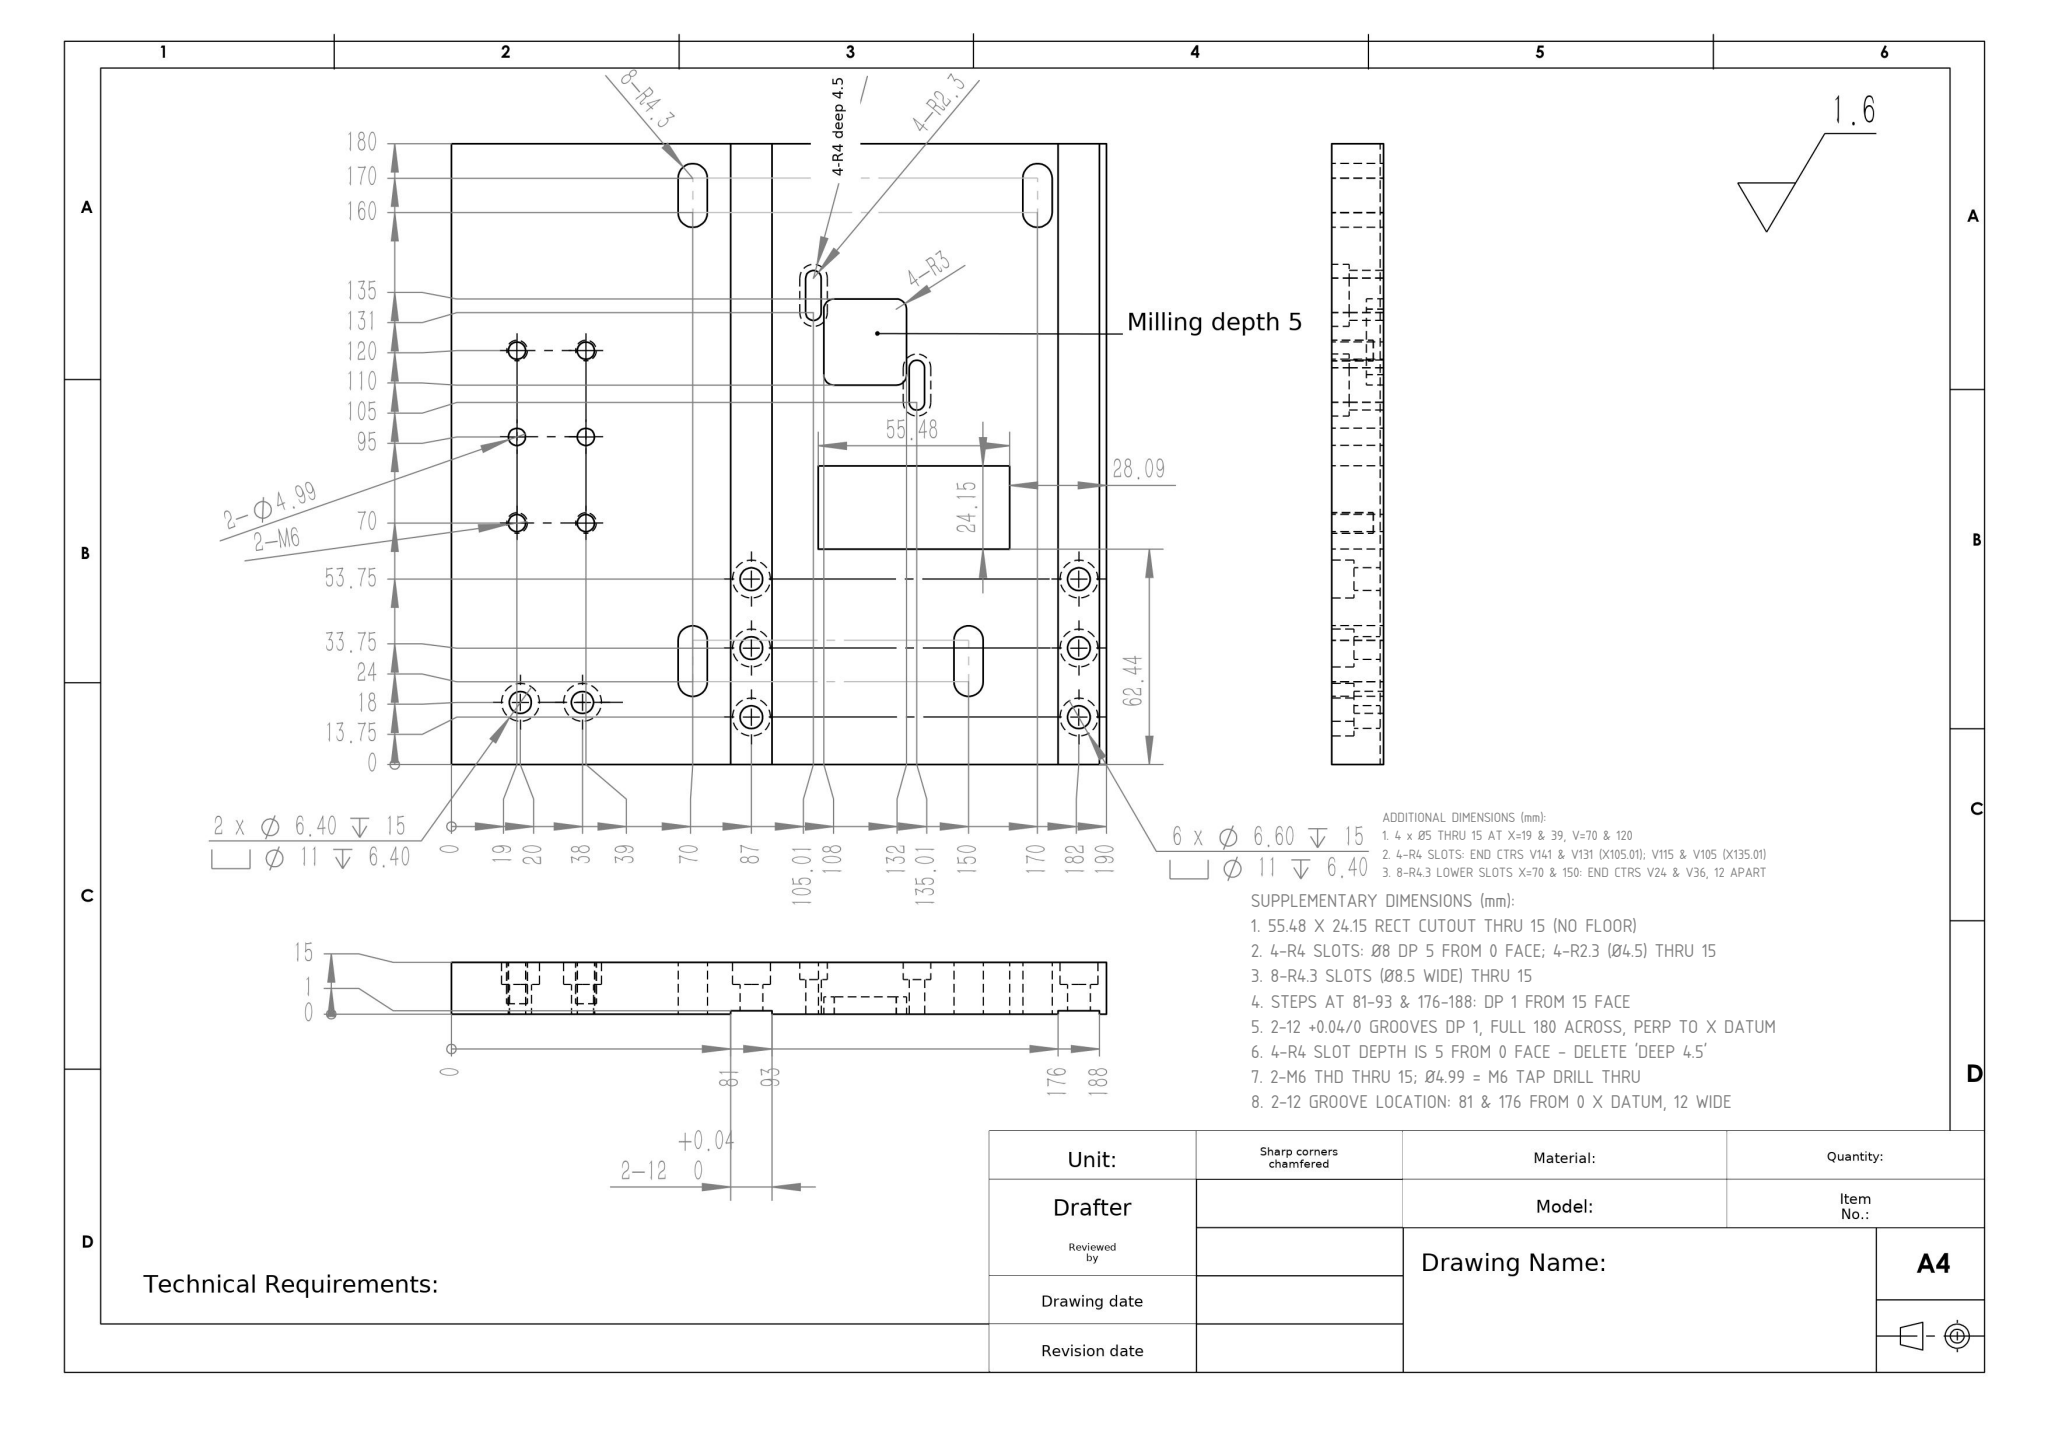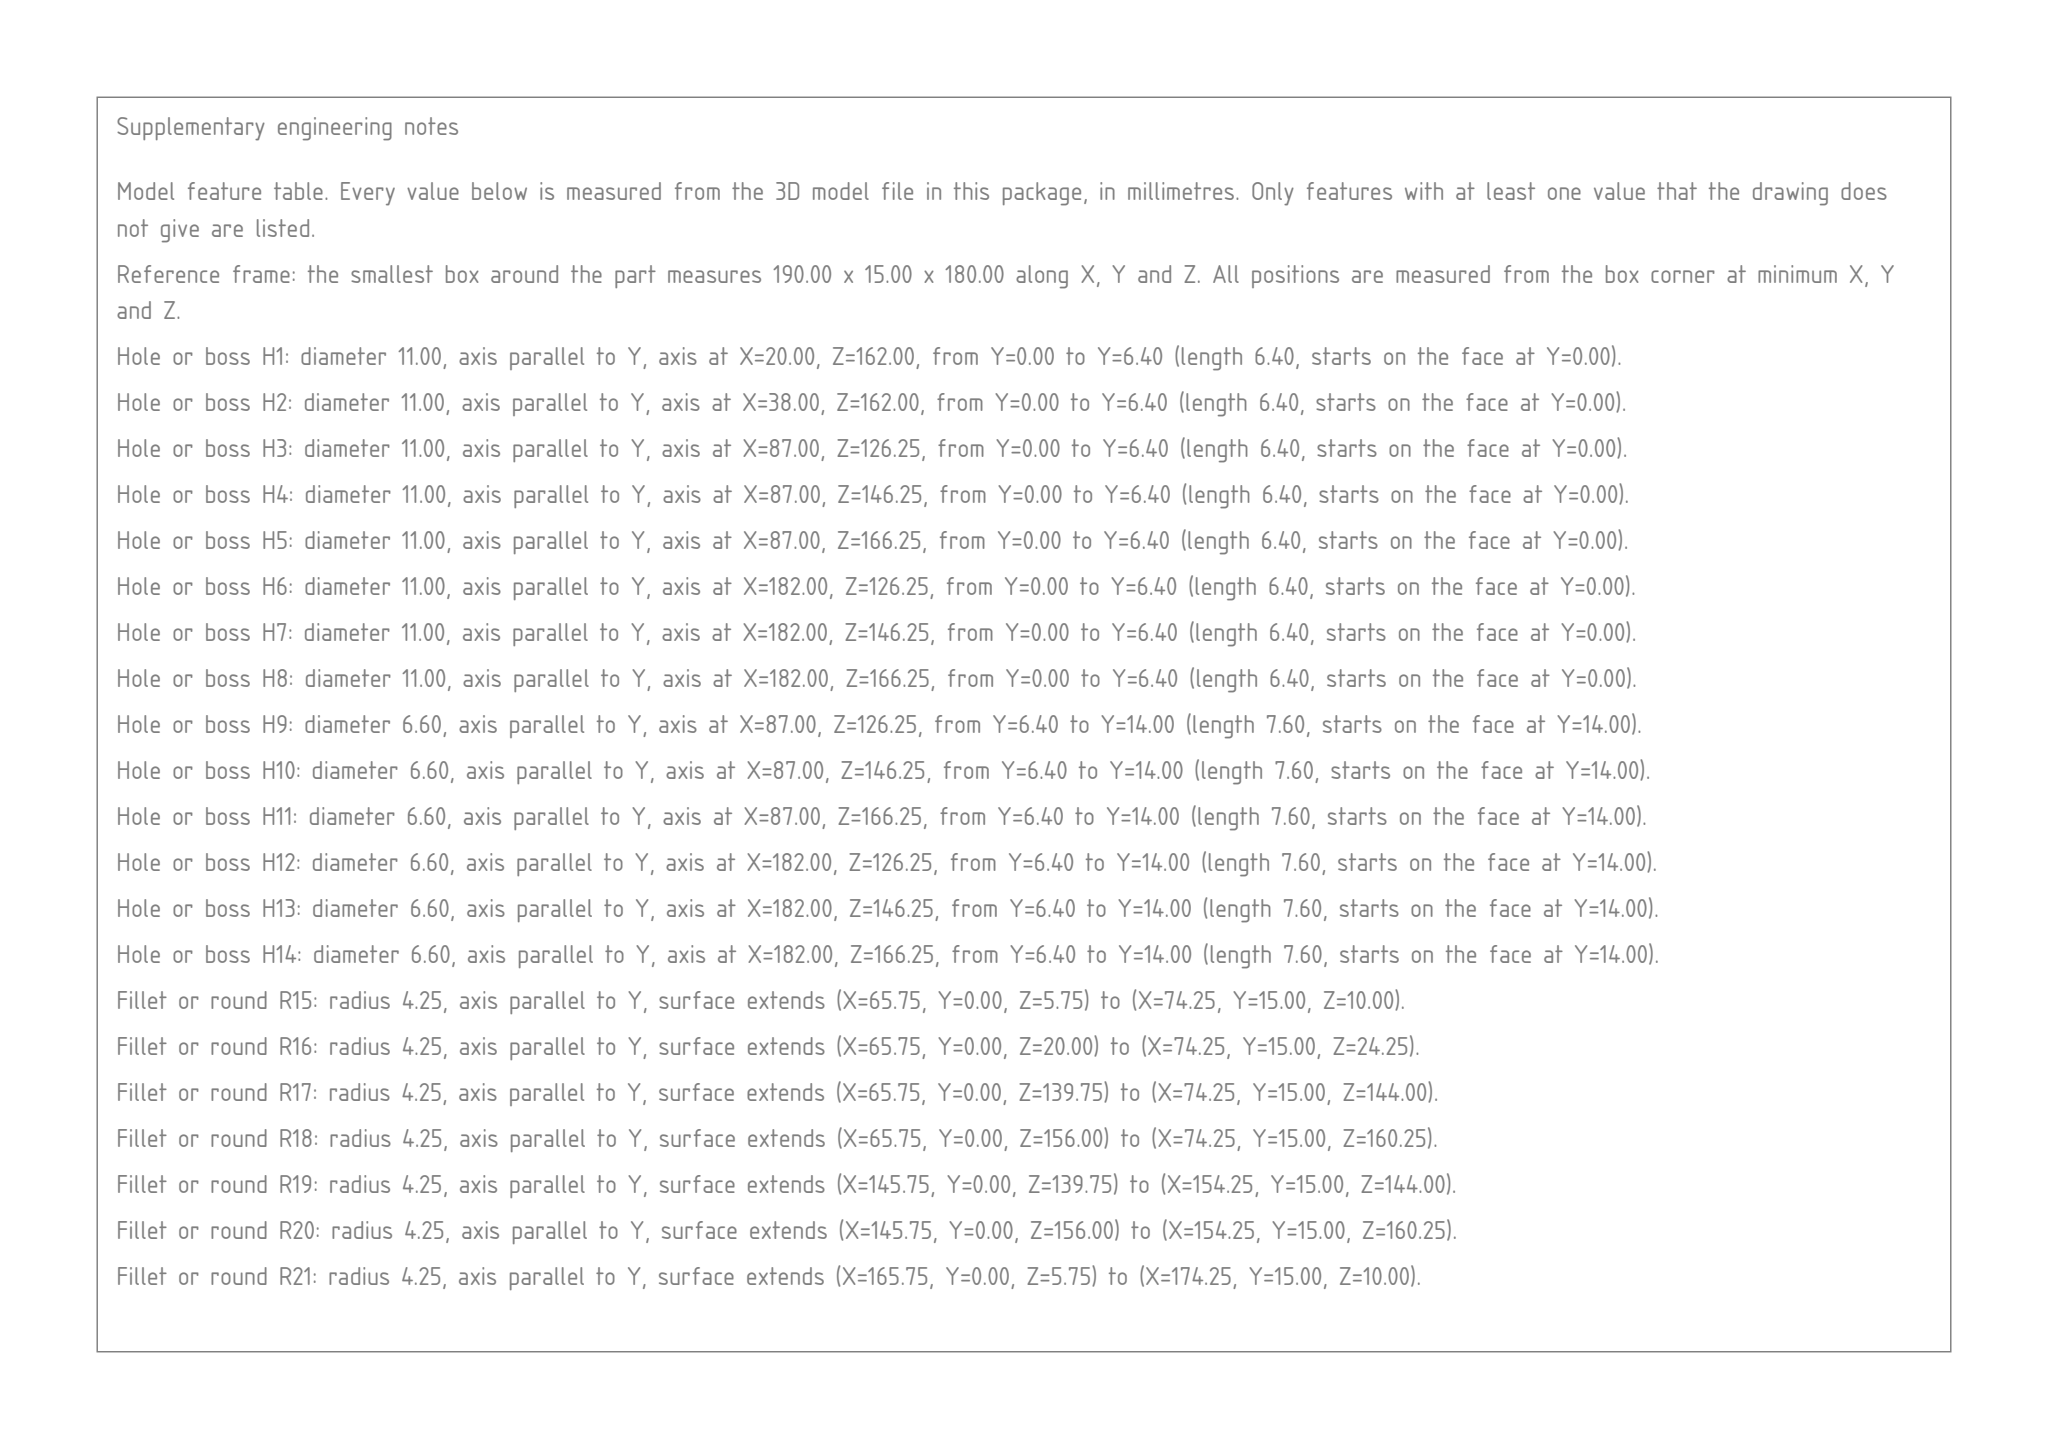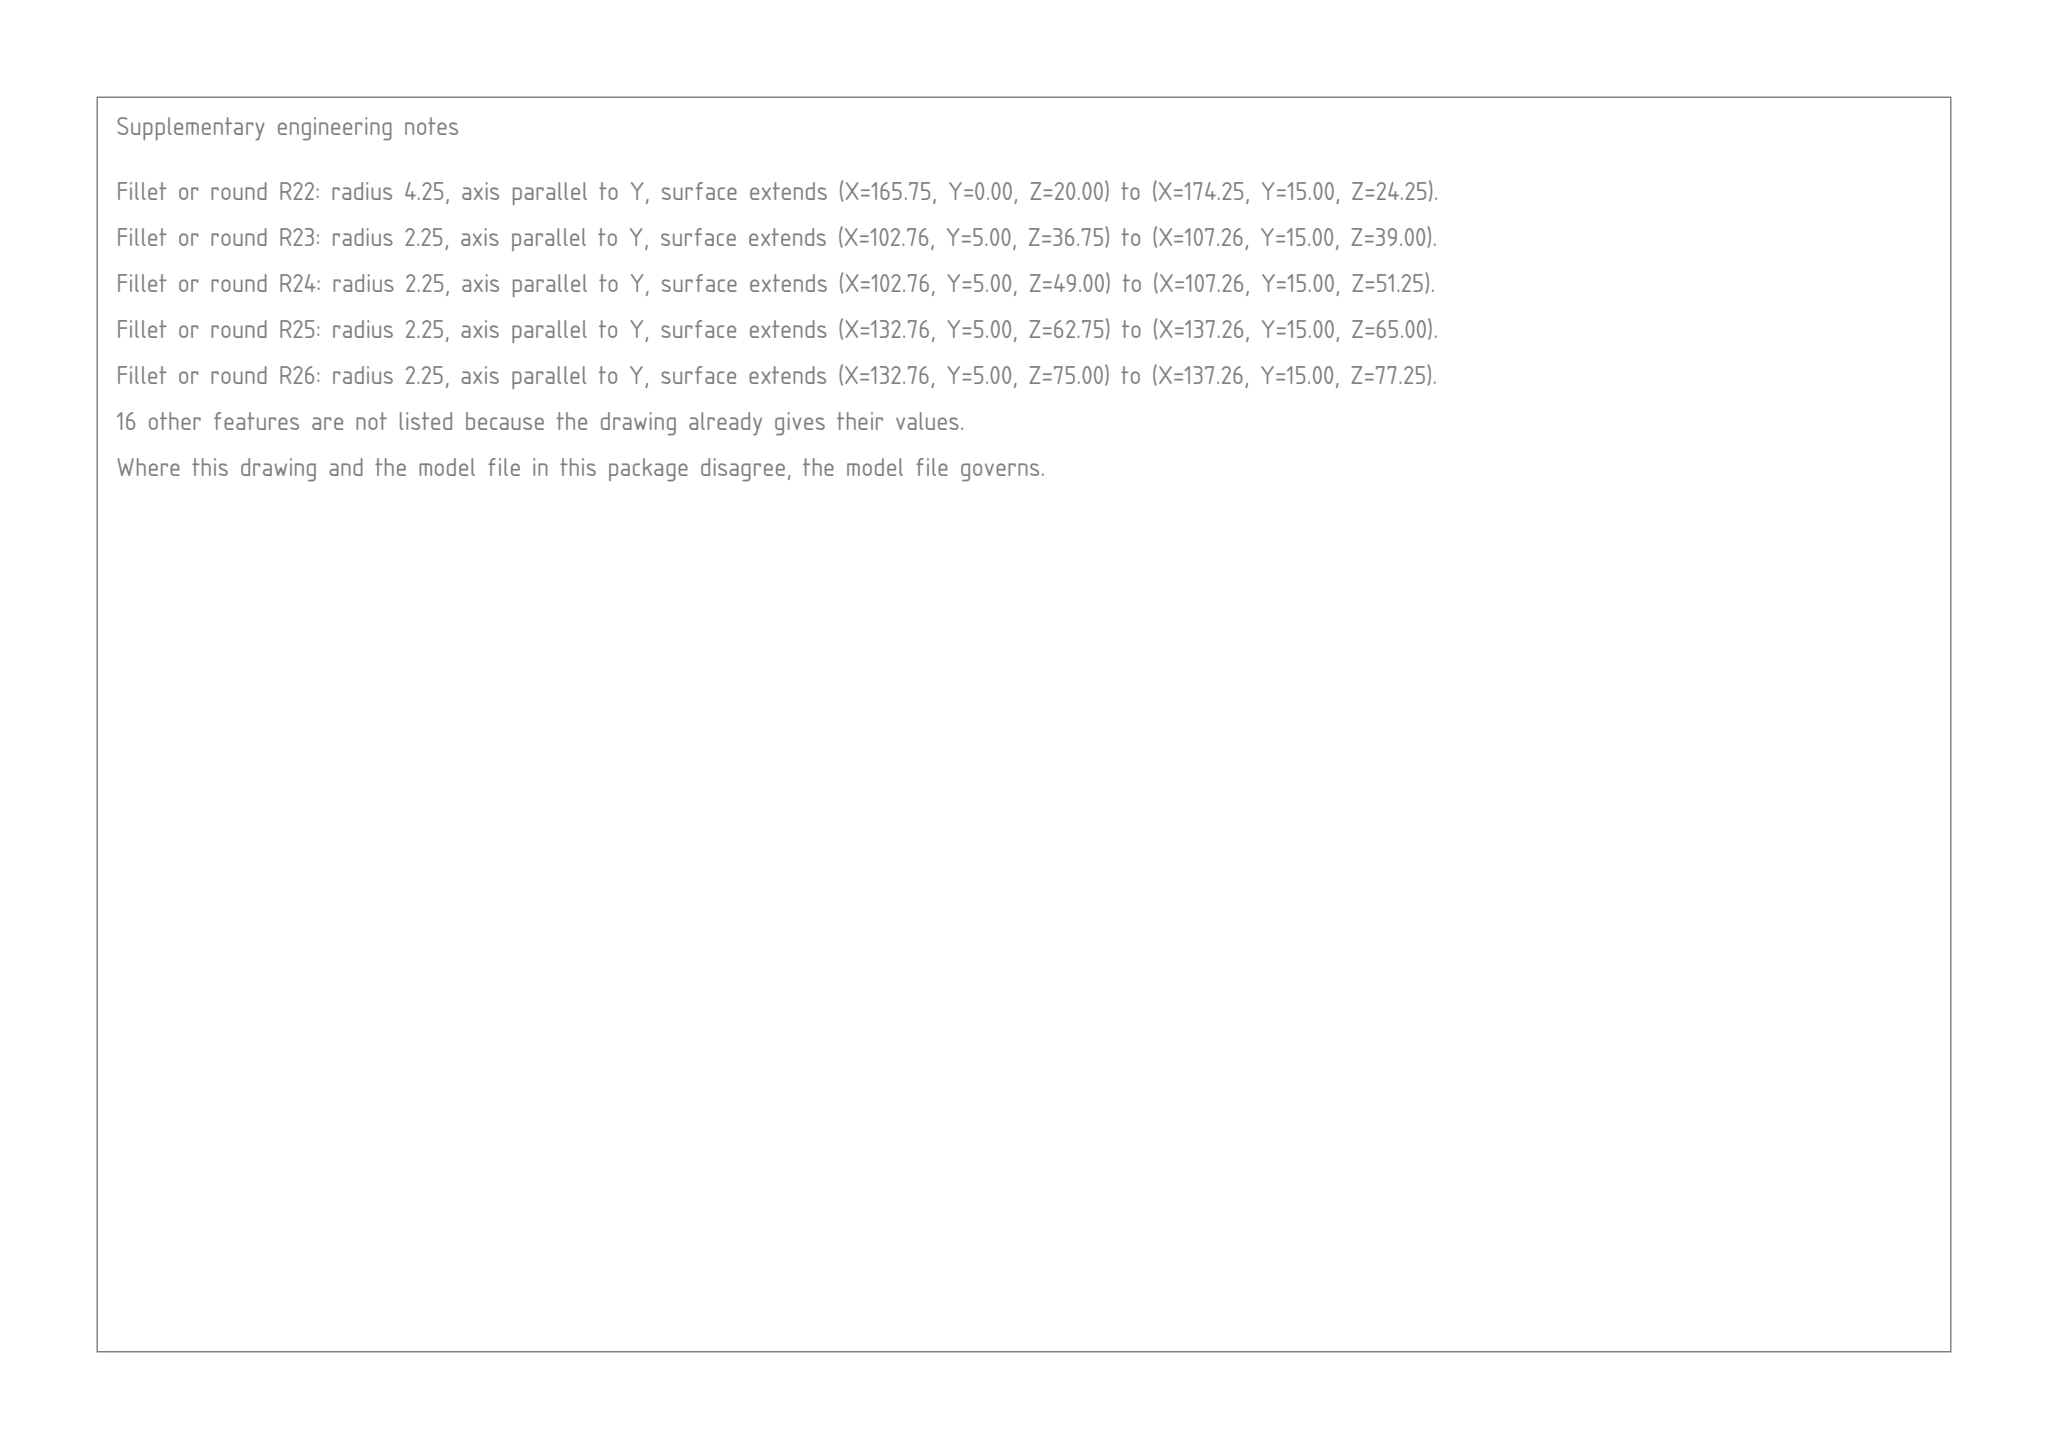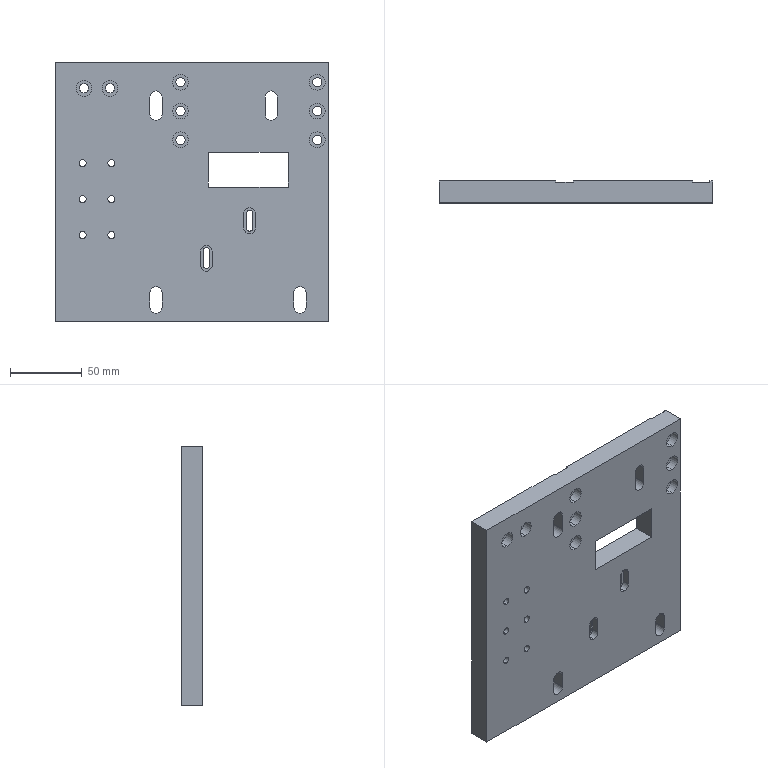Part | SolidWorks | mm | 1 solid | 121 faces | box 190 x 15 x 180 mm | volume 465345 mm3 | cylinder 72 | plane 49 | commonest cylinder face diameters 11 x16 6.6 x12 8.5 x12 5 x8 8 x6 4.5 x6 6.4 x4 4.99 x4
build123d program:
from build123d import *

# Parameters (mm, degrees)
SKETCH1_W                                       = 190
SKETCH1_H                                       = 180
BOSS_EXTRUDE1_DEPTH                             = 15
CUT_EXTRUDE2_DEPTH                              = 24
M6_TAPPED_HOLE1_D                               = 5
M6_TAPPED_HOLE1_DEPTH                           = 15
M6_TAPPED_HOLE1_TIP                             = 1.502
M4_HEX_SOCKET_HEAD_CAP_SCREW_CBORE1_D           = 4.5
M4_HEX_SOCKET_HEAD_CAP_SCREW_CBORE1_DEPTH       = 15
M4_HEX_SOCKET_HEAD_CAP_SCREW_CBORE1_CBORE_D     = 8
M4_HEX_SOCKET_HEAD_CAP_SCREW_CBORE1_CBORE_DEPTH = 4.4
M4_HEX_SOCKET_HEAD_CAP_SCREW_CBORE1_TIP         = 1.352
M6_HEX_SOCKET_HEAD_CAP_SCREW_CBORE1_D           = 6.6
M6_HEX_SOCKET_HEAD_CAP_SCREW_CBORE1_DEPTH       = 15
M6_HEX_SOCKET_HEAD_CAP_SCREW_CBORE1_CBORE_D     = 11
M6_HEX_SOCKET_HEAD_CAP_SCREW_CBORE1_CBORE_DEPTH = 6.4
M6_HEX_SOCKET_HEAD_CAP_SCREW_CBORE1_TIP         = 1.983
F_5_0_5_DIAMETER_HOLE1_D                        = 4.99
M6_HEX_SOCKET_HEAD_CAP_SCREW_CBORE2_D           = 6.4
M6_HEX_SOCKET_HEAD_CAP_SCREW_CBORE2_DEPTH       = 15
M6_HEX_SOCKET_HEAD_CAP_SCREW_CBORE2_CBORE_D     = 11
M6_HEX_SOCKET_HEAD_CAP_SCREW_CBORE2_CBORE_DEPTH = 6.4
M6_HEX_SOCKET_HEAD_CAP_SCREW_CBORE2_TIP         = 1.923
CUT_EXTRUDE3_DEPTH                              = 263.155
CUT_EXTRUDE4_DEPTH                              = 5
CUT_EXTRUDE5_DEPTH                              = 263.155
CUT_EXTRUDE6_DEPTH                              = 5
SKETCH24_W                                      = 24
SKETCH24_H                                      = 25
CUT_EXTRUDE7_DEPTH                              = 5
FILLET1_R                                       = 3
SKETCH25_W                                      = 12
SKETCH25_H                                      = 1
CUT_EXTRUDE8_DEPTH                              = 263.155
SKETCH26_W                                      = 55.48
SKETCH26_H                                      = 24.146
CUT_EXTRUDE9_DEPTH                              = 61


with BuildPart() as part:
    # Sketch1 → Boss-Extrude1 (new body)
    with BuildSketch(Plane(origin=(0, 0, 0), x_dir=(1, 0, 0), z_dir=(0, 1, 0))):
        with Locations((95, 90)):
            Rectangle(SKETCH1_W, SKETCH1_H)
    extrude(amount=BOSS_EXTRUDE1_DEPTH)

    # Sketch6 → Cut-Extrude2 (cut)
    with BuildSketch(Plane(origin=(0, 15, 0), x_dir=(-1, 0, 0), z_dir=(0, 1, 0))):
        with BuildLine():
            Line((-165.75, -160), (-165.75, -170))
            ThreePointArc((-165.75, -170), (-170, -174.25), (-174.25, -170))
            Line((-174.25, -170), (-174.25, -160))
            ThreePointArc((-174.25, -160), (-170, -155.75), (-165.75, -160))
        make_face()
        with BuildLine():
            Line((-65.75, -160), (-65.75, -170))
            ThreePointArc((-65.75, -170), (-70, -174.25), (-74.25, -170))
            Line((-74.25, -170), (-74.25, -160))
            ThreePointArc((-74.25, -160), (-70, -155.75), (-65.75, -160))
        make_face()
        with BuildLine():
            Line((-145.75, -24), (-145.75, -36))
            ThreePointArc((-145.75, -36), (-150, -40.25), (-154.25, -36))
            Line((-154.25, -36), (-154.25, -24))
            ThreePointArc((-154.25, -24), (-150, -19.75), (-145.75, -24))
        make_face()
        with BuildLine():
            Line((-65.75, -24), (-65.75, -36))
            ThreePointArc((-65.75, -36), (-70, -40.25), (-74.25, -36))
            Line((-74.25, -36), (-74.25, -24))
            ThreePointArc((-74.25, -24), (-70, -19.75), (-65.75, -24))
        make_face()
    extrude(amount=-CUT_EXTRUDE2_DEPTH, mode=Mode.SUBTRACT)

    # M6 Tapped Hole1
    with Locations(Plane(origin=(0, 0, 0), x_dir=(-1, 0, 0), z_dir=(0, -1, 0))):
        with Locations((-39, 70), (-19, 120), (-39, 120), (-19, 70)):
            Hole(M6_TAPPED_HOLE1_D / 2, depth=M6_TAPPED_HOLE1_DEPTH)
            with Locations((0, 0, -(M6_TAPPED_HOLE1_DEPTH + M6_TAPPED_HOLE1_TIP / 2))):  # 118° drill point
                Cone(0, M6_TAPPED_HOLE1_D / 2, M6_TAPPED_HOLE1_TIP, mode=Mode.SUBTRACT)

    # M4 Hex Socket Head Cap Screw CBORE1
    with Locations(Plane(origin=(105.01, 0, -136.3), x_dir=(0, 0, -1), z_dir=(0, -1, 0))):
        with Locations((0, 0), (-26, 30)):
            CounterBoreHole(M4_HEX_SOCKET_HEAD_CAP_SCREW_CBORE1_D / 2, M4_HEX_SOCKET_HEAD_CAP_SCREW_CBORE1_CBORE_D / 2, M4_HEX_SOCKET_HEAD_CAP_SCREW_CBORE1_CBORE_DEPTH, depth=M4_HEX_SOCKET_HEAD_CAP_SCREW_CBORE1_DEPTH)
            with Locations((0, 0, -(M4_HEX_SOCKET_HEAD_CAP_SCREW_CBORE1_DEPTH + M4_HEX_SOCKET_HEAD_CAP_SCREW_CBORE1_TIP / 2))):  # 118° drill point
                Cone(0, M4_HEX_SOCKET_HEAD_CAP_SCREW_CBORE1_D / 2, M4_HEX_SOCKET_HEAD_CAP_SCREW_CBORE1_TIP, mode=Mode.SUBTRACT)

    # M6 Hex Socket Head Cap Screw CBORE1
    with Locations(Plane(origin=(182, 0, -53.75), x_dir=(0, 0, -1), z_dir=(0, -1, 0))):
        with Locations((0, 0), (-20, 0), (-40, 0), (0, -95), (-20, -95), (-40, -95)):
            CounterBoreHole(M6_HEX_SOCKET_HEAD_CAP_SCREW_CBORE1_D / 2, M6_HEX_SOCKET_HEAD_CAP_SCREW_CBORE1_CBORE_D / 2, M6_HEX_SOCKET_HEAD_CAP_SCREW_CBORE1_CBORE_DEPTH, depth=M6_HEX_SOCKET_HEAD_CAP_SCREW_CBORE1_DEPTH)
            with Locations((0, 0, -(M6_HEX_SOCKET_HEAD_CAP_SCREW_CBORE1_DEPTH + M6_HEX_SOCKET_HEAD_CAP_SCREW_CBORE1_TIP / 2))):  # 118° drill point
                Cone(0, M6_HEX_SOCKET_HEAD_CAP_SCREW_CBORE1_D / 2, M6_HEX_SOCKET_HEAD_CAP_SCREW_CBORE1_TIP, mode=Mode.SUBTRACT)

    # 5.0 _5_ Diameter Hole1 (through all)
    with Locations(Plane(origin=(19, 0, -95), x_dir=(0, 0, -1), z_dir=(0, -1, 0))):
        with Locations((0, 0), (0, 20)):
            Hole(F_5_0_5_DIAMETER_HOLE1_D / 2)

    # M6 Hex Socket Head Cap Screw CBORE2
    with Locations(Plane(origin=(38, 0, -18), x_dir=(0, 0, -1), z_dir=(0, -1, 0))):
        with Locations((0, 0), (0, -18)):
            CounterBoreHole(M6_HEX_SOCKET_HEAD_CAP_SCREW_CBORE2_D / 2, M6_HEX_SOCKET_HEAD_CAP_SCREW_CBORE2_CBORE_D / 2, M6_HEX_SOCKET_HEAD_CAP_SCREW_CBORE2_CBORE_DEPTH, depth=M6_HEX_SOCKET_HEAD_CAP_SCREW_CBORE2_DEPTH)
            with Locations((0, 0, -(M6_HEX_SOCKET_HEAD_CAP_SCREW_CBORE2_DEPTH + M6_HEX_SOCKET_HEAD_CAP_SCREW_CBORE2_TIP / 2))):  # 118° drill point
                Cone(0, M6_HEX_SOCKET_HEAD_CAP_SCREW_CBORE2_D / 2, M6_HEX_SOCKET_HEAD_CAP_SCREW_CBORE2_TIP, mode=Mode.SUBTRACT)

    # Sketch20 → Cut-Extrude3 (cut, through all)
    with BuildSketch(Plane.XZ):
        with BuildLine():
            Line((137.26, -105), (137.26, -115))
            ThreePointArc((137.26, -115), (135.01, -117.25), (132.76, -115))
            Line((132.76, -115), (132.76, -105))
            ThreePointArc((132.76, -105), (135.01, -102.75), (137.26, -105))
        make_face()
    extrude(amount=-CUT_EXTRUDE3_DEPTH, mode=Mode.SUBTRACT)

    # Sketch21 → Cut-Extrude4 (cut)
    with BuildSketch(Plane.XZ):
        with BuildLine():
            Line((139.01, -105), (139.01, -115))
            ThreePointArc((139.01, -115), (135.01, -119), (131.01, -115))
            Line((131.01, -115), (131.01, -105))
            ThreePointArc((131.01, -105), (135.01, -101), (139.01, -105))
        make_face()
    extrude(amount=-CUT_EXTRUDE4_DEPTH, mode=Mode.SUBTRACT)

    # Sketch22 → Cut-Extrude5 (cut, through all)
    with BuildSketch(Plane.XZ):
        with BuildLine():
            Line((107.26, -131), (107.26, -141))
            ThreePointArc((107.26, -141), (105.01, -143.25), (102.76, -141))
            Line((102.76, -141), (102.76, -131))
            ThreePointArc((102.76, -131), (105.01, -128.75), (107.26, -131))
        make_face()
    extrude(amount=-CUT_EXTRUDE5_DEPTH, mode=Mode.SUBTRACT)

    # Sketch23 → Cut-Extrude6 (cut)
    with BuildSketch(Plane.XZ):
        with BuildLine():
            Line((101.01, -141), (101.01, -131))
            ThreePointArc((101.01, -131), (105.01, -127), (109.01, -131))
            Line((109.01, -131), (109.01, -141))
            ThreePointArc((109.01, -141), (105.01, -145), (101.01, -141))
        make_face()
    extrude(amount=-CUT_EXTRUDE6_DEPTH, mode=Mode.SUBTRACT)

    # Sketch24 → Cut-Extrude7 (cut)
    with BuildSketch(Plane(origin=(0, 15, 0), x_dir=(1, 0, 0), z_dir=(0, 1, 0))):
        with Locations((120, 122.5)):
            Rectangle(SKETCH24_W, SKETCH24_H)
    extrude(amount=-CUT_EXTRUDE7_DEPTH, mode=Mode.SUBTRACT)

    # Fillet1
    fillet1_edges = [part.edges().sort_by_distance(p)[0] for p in [
        (108, 12.5, -110),
        (108, 12.5, -135),
        (132, 12.5, -135),
        (132, 12.5, -110),
    ]]
    fillet(fillet1_edges, radius=FILLET1_R)

    # Sketch25 → Cut-Extrude8 (cut, through all)
    with BuildSketch(Plane.XY):
        with Locations((182, 14.5)):
            Rectangle(SKETCH25_W, SKETCH25_H)
        with Locations((87, 14.5)):
            Rectangle(SKETCH25_W, SKETCH25_H)
    extrude(amount=-CUT_EXTRUDE8_DEPTH, mode=Mode.SUBTRACT)

    # Sketch26 → Cut-Extrude9 (cut)
    with BuildSketch(Plane(origin=(0, 15, 0), x_dir=(1, 0, 0), z_dir=(0, 1, 0))):
        with Locations((134.168, 74.517)):
            Rectangle(SKETCH26_W, SKETCH26_H)
    extrude(amount=-CUT_EXTRUDE9_DEPTH, mode=Mode.SUBTRACT)


solid = part.part